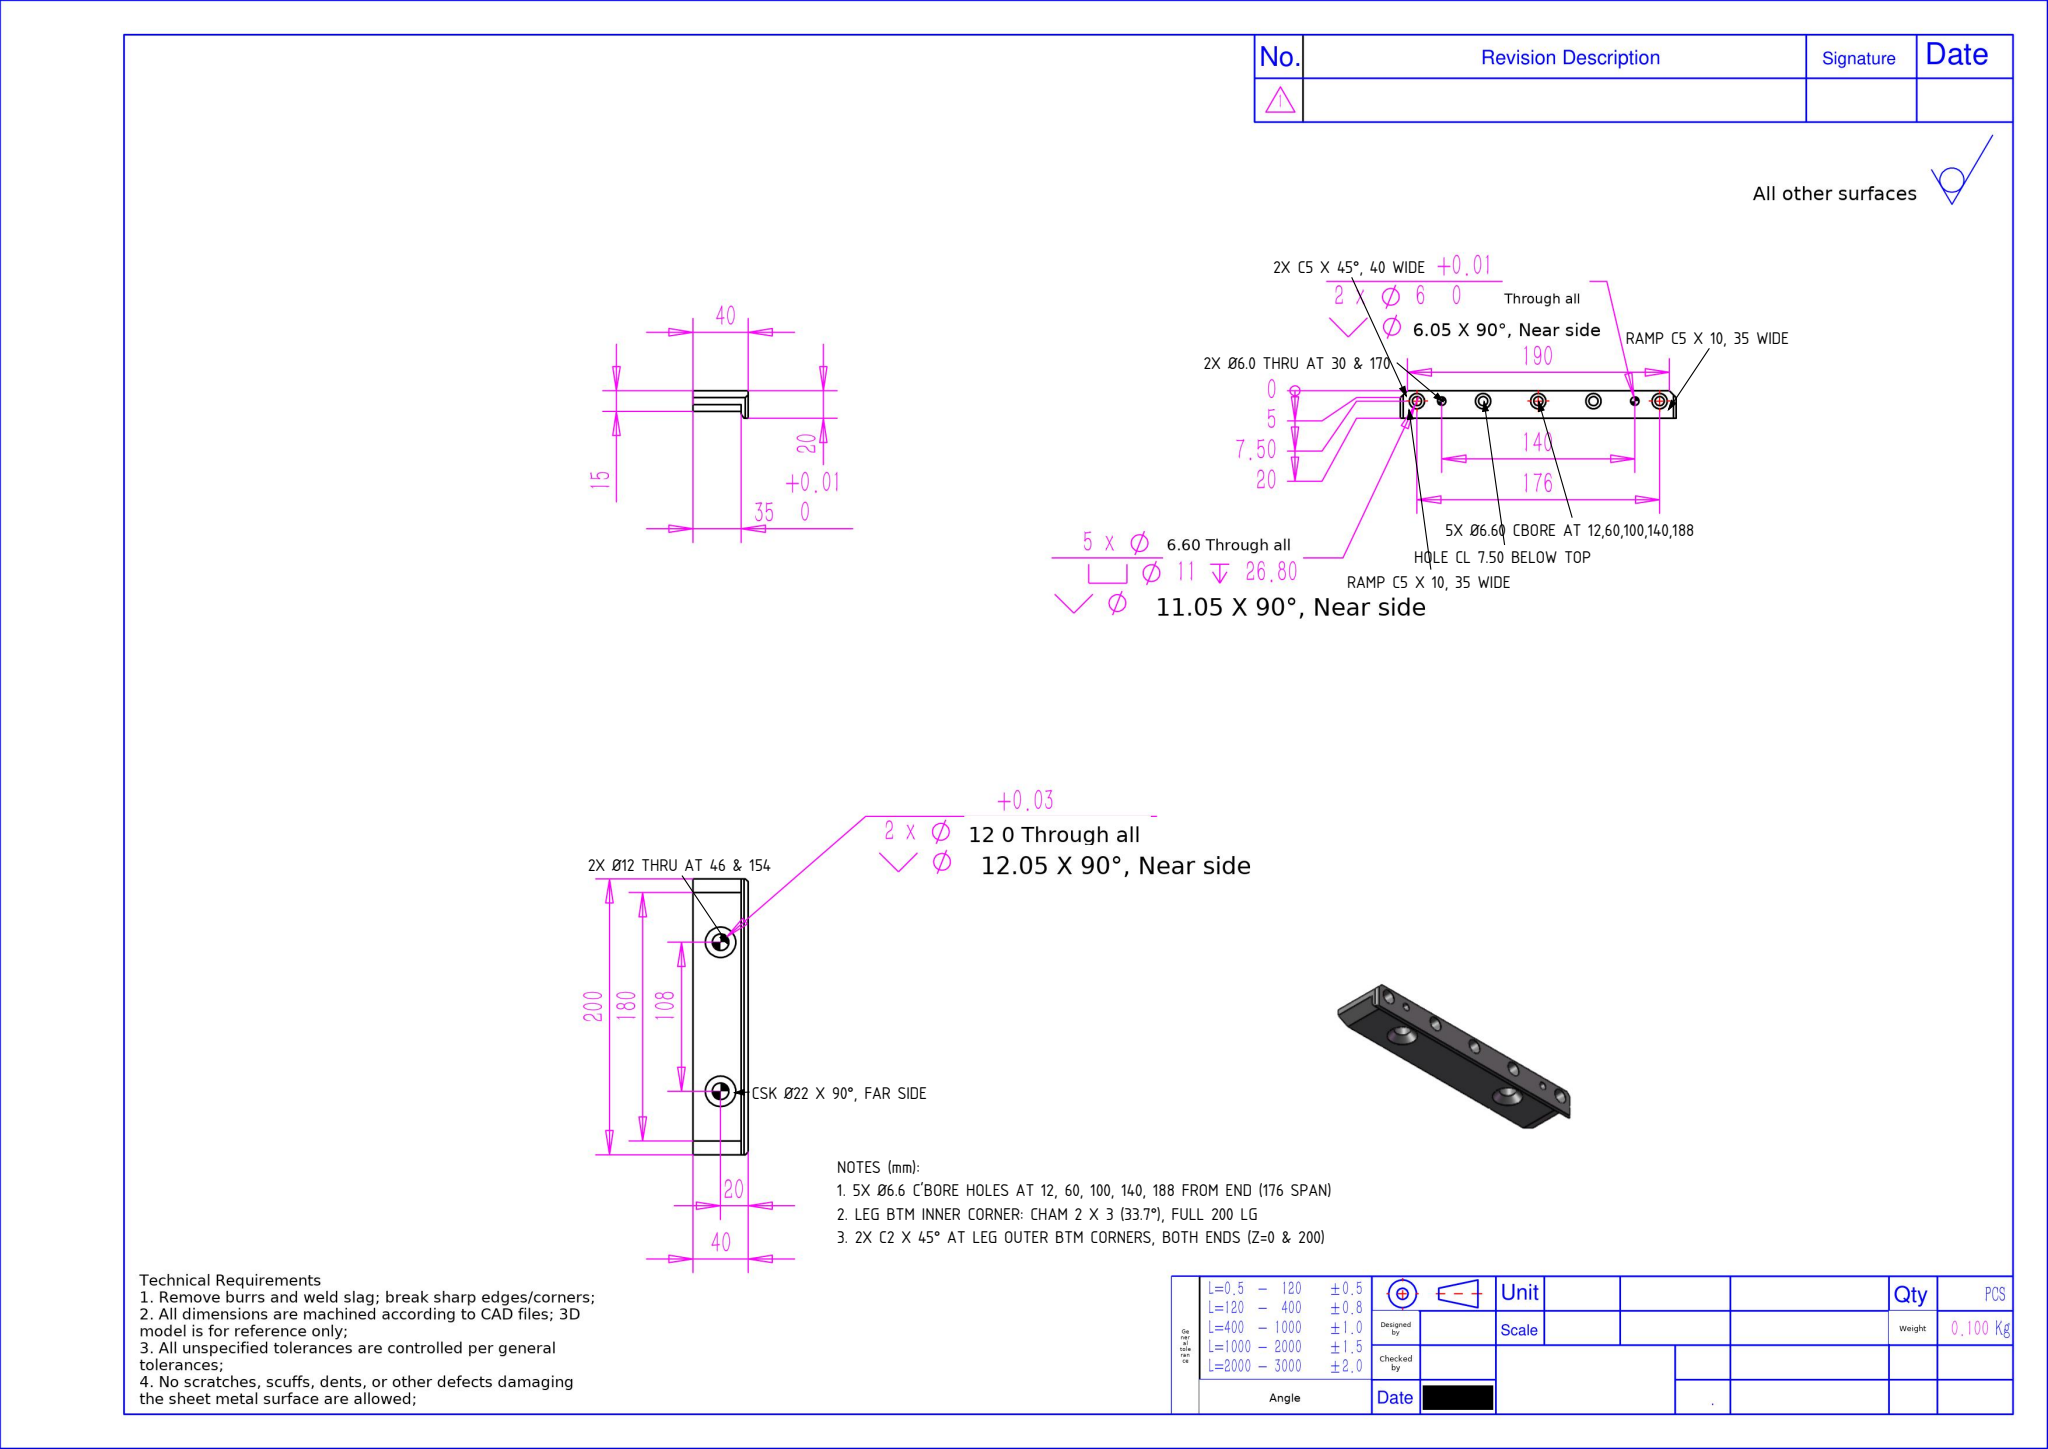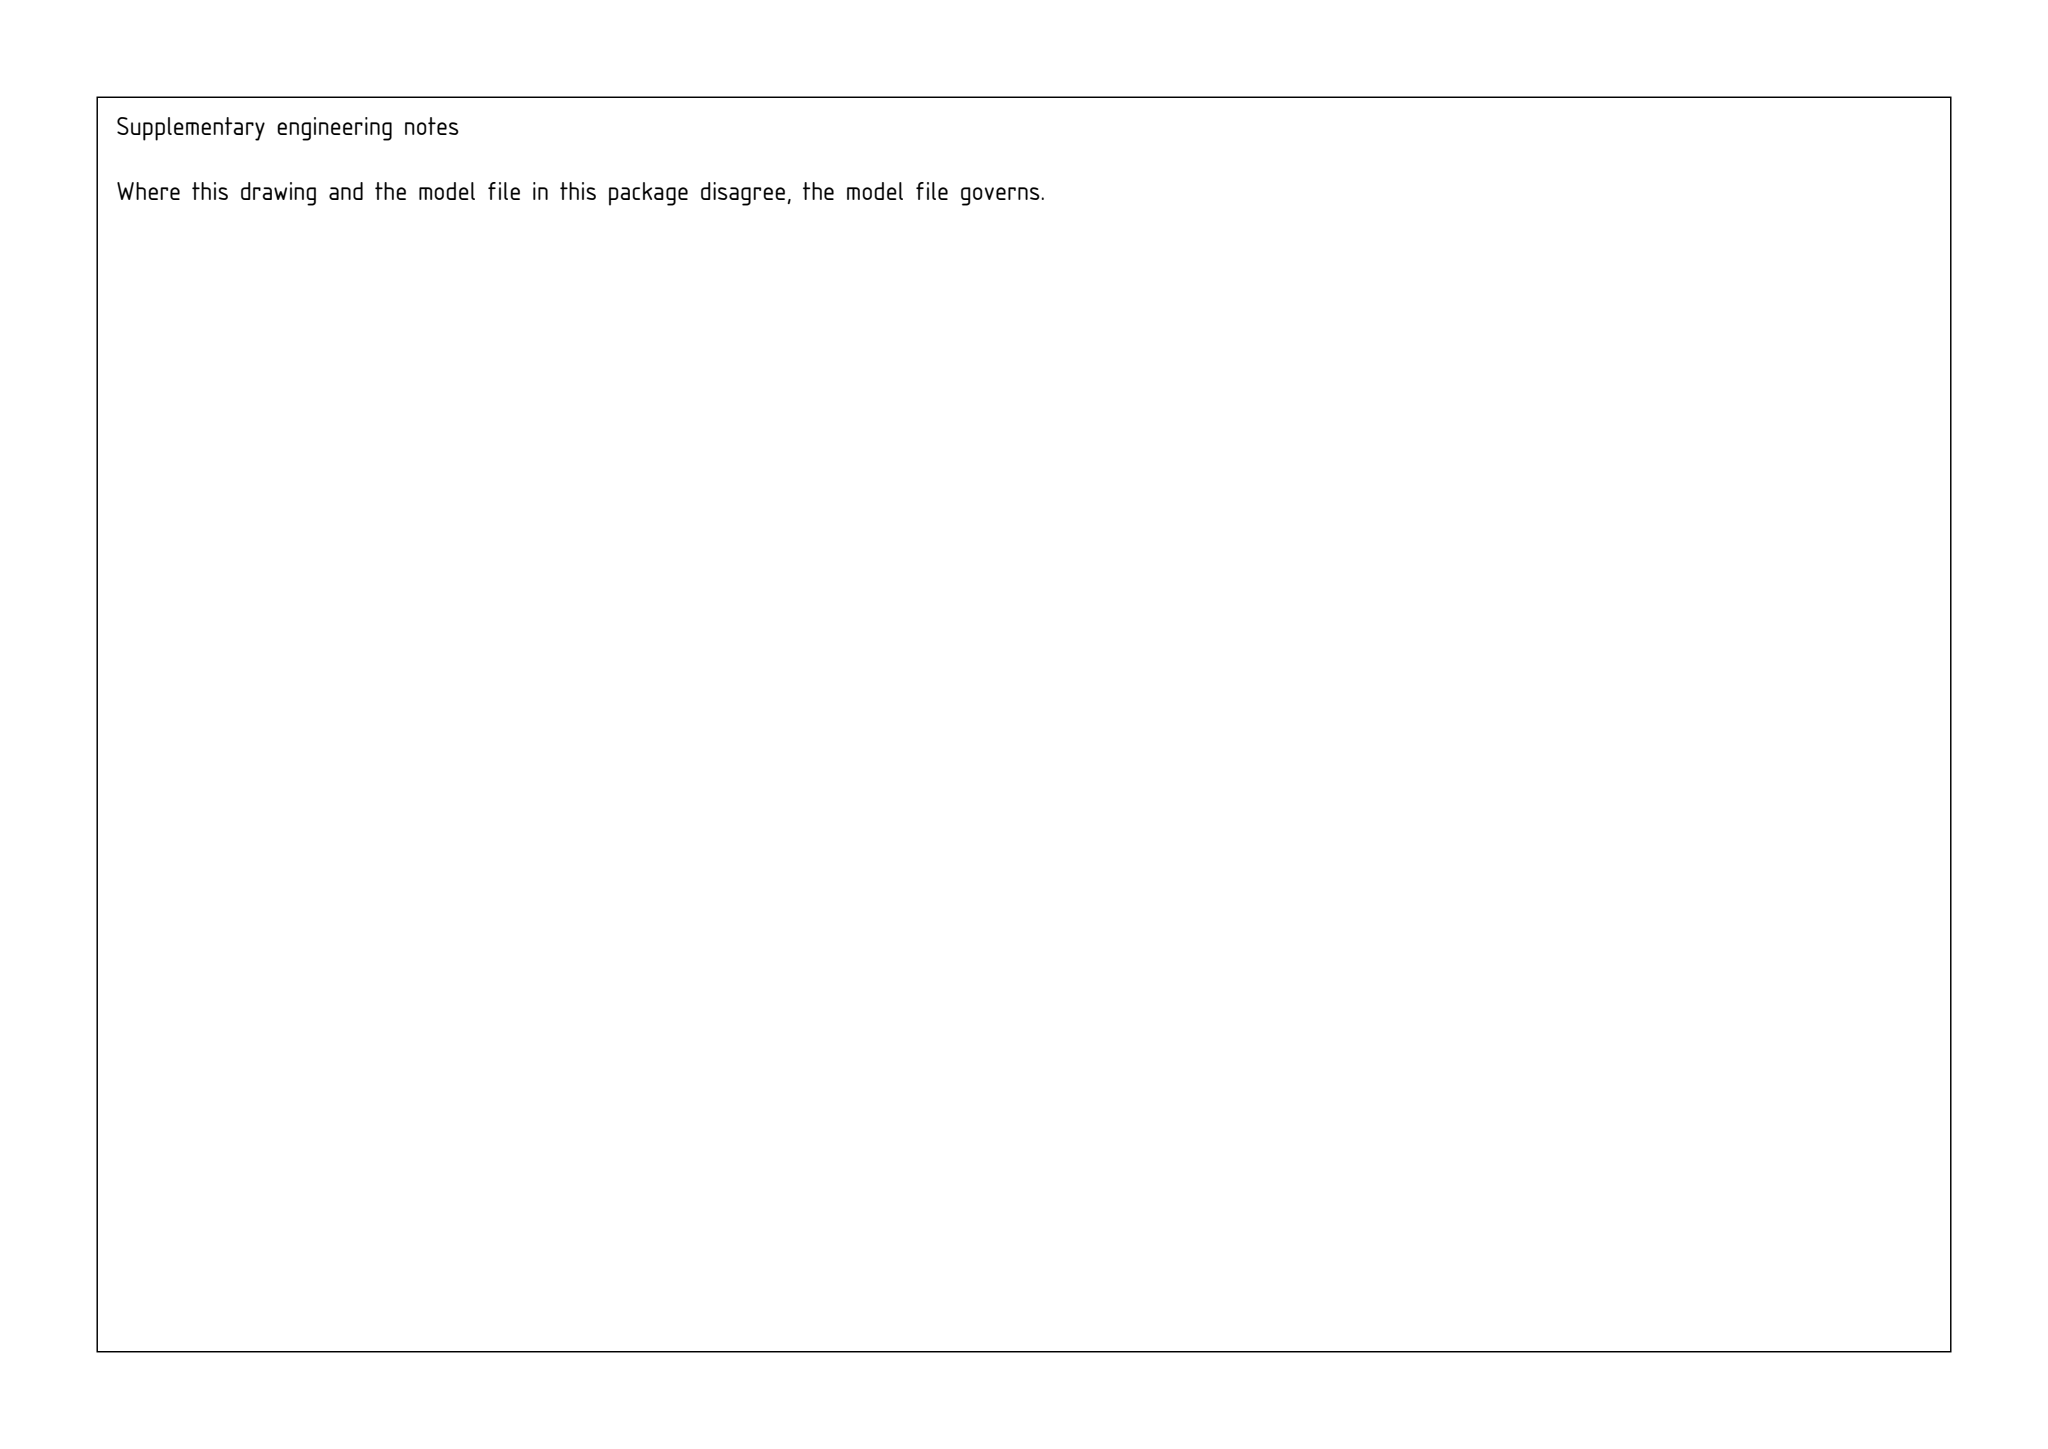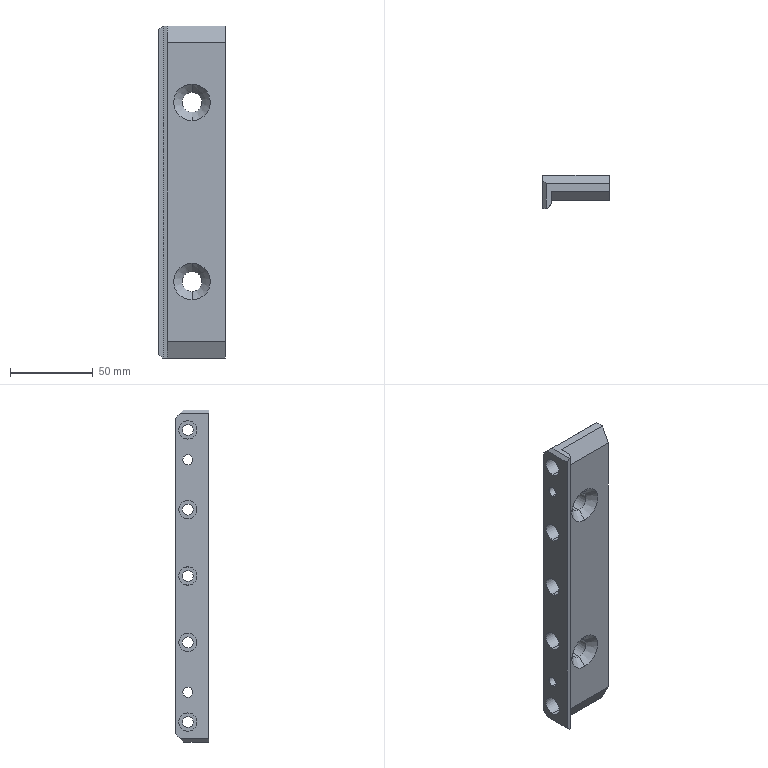Part | SolidWorks | mm | 1 solid | 70 faces | box 40 x 20 x 200 mm | volume 99736 mm3 | cylinder 28 | cone 22 | plane 20 | commonest cylinder face diameters 11 x10 6.6 x10 6 x4 12 x4
Drawing notes:
5X Ø6.60 CBORE HOLES AT 12, 60, 100, 140, 188 FROM LH END | from the solid: Ø6.6/Ø11 x-axis cyls at z = 12.0, 60.0, 100.0, 140.0, 188.0 of 200 lg
2X Ø6.0 THRU AT 30 & 170 FROM LH END | from the solid: Ø6.0 cyls, axis x, z = 30.0 and 170.0
ALL Ø6.60 & Ø6.0 HOLE CL 12.50 ABV BASE (7.50 BELOW TOP) | from the solid: all x-axis cyls at y = 12.5; y planes at 0, 5, 20
2X Ø12.0 THRU AT 46 & 154 FROM LH END, CL 20 FROM SIDE FACE | from the solid: Ø12.0 cyls, axis y, pos [20.0, null, 46.0] and [20.0, null, 154.0]
5X Ø6.6 C'BORE HOLES AT 12, 60, 100, 140, 188 FROM END (176 SPAN) | from the solid: Ø6.6/Ø11 bores at z=12,60,100,140,188; y=12.5; outer span 188-12=176
2X Ø12 THRU: ADD C'SINK Ø22 X 90°, FAR SIDE (FLANGE UNDERSIDE) | from the solid: cones 90°, ref_dia 12.0, from y=5 to y=10, size [11,5,22] at z=35 & 143
LEG BTM INNER CORNER: CHAM 2 X 3 (33.7°), FULL 200 LG | from the solid: inclined plane angles [33.7,56.3,90], from [3,0,0], size [2,3,200]
2X C2 X 45° AT LEG OUTER BTM CORNERS, BOTH ENDS (Z=0 & 200) | from the solid: inclined planes 45°, from [0,0,0] & [0,0,198], size [2,17,2]
2X C5 X 45° AT TOP EDGE OF BOTH END FACES, 40 WIDE | from the solid: inclined planes 45°, from [0,15,0] & [0,15,195], size [40,5,5]
FLANGE UNDERSIDE RAMP BOTH ENDS: 5 RISE X 10 RUN (26.6°), 35 WIDE | from the solid: inclined planes [90,26.6,63.4], from [5,5,0] & [5,5,190], size [35,5,10]
2X RAMP C5 X 10, 35 WIDE, BOTH ENDS OF 200 LG | from the solid: inclined_planes [90,26.6,63.4] at bbox_from [5,5,0] and [5,5,190], size [35,5,10] each
build123d program:
from build123d import *

# Parameters (mm, degrees)
BOSS_EXTRUDE1_DEPTH                            = 100
CHAMFER1_SIZE                                  = 2
M6_HEX_SOCKET_HEAD_CAP_SCREW_CBORE1_AT_2_COUNT = 2
M6_HEX_SOCKET_HEAD_CAP_SCREW_CBORE1_AT_2_PITCH = 88
M6_HEX_SOCKET_HEAD_CAP_SCREW_CBORE1_AT_3_COUNT = 2
M6_HEX_SOCKET_HEAD_CAP_SCREW_CBORE1_AT_3_PITCH = 176
M6_HEX_SOCKET_HEAD_CAP_SCREW_CBORE1_AT_4_COUNT = 2
M6_HEX_SOCKET_HEAD_CAP_SCREW_CBORE1_AT_4_PITCH = 48
M6_HEX_SOCKET_HEAD_CAP_SCREW_CBORE1_AT_5_COUNT = 2
M6_HEX_SOCKET_HEAD_CAP_SCREW_CBORE1_AT_5_PITCH = 128
F_12_0MM_DOWEL_PIN_HOLE1_D                     = 12
F_12_0MM_DOWEL_PIN_HOLE1_CSINK_D               = 12.05
F_12_0MM_DOWEL_PIN_HOLE1_CSINK_ANGLE           = 90
CHAMFER2_SIZE                                  = 5
CHAMFER2_SIZE2                                 = 10
F_6_0MM_DOWEL_PIN_HOLE1_D                      = 6
F_6_0MM_DOWEL_PIN_HOLE1_CSINK_D                = 6.05
F_6_0MM_DOWEL_PIN_HOLE1_CSINK_ANGLE            = 90
CHAMFER3_SIZE                                  = 10
CHAMFER3_SIZE2                                 = 5
CHAMFER4_SIZE                                  = 2
CHAMFER4_SIZE2                                 = 3
CHAMFER5_SIZE                                  = 5
CHAMFER6_SIZE                                  = 5


with BuildPart() as part:
    # Sketch1 → Boss-Extrude1 (new, symmetric)
    with BuildSketch(Plane.XY):
        Polygon((40, 0), (0, 0), (0, -20), (5, -20), (5, -15), (40, -15), align=None)
    extrude(amount=BOSS_EXTRUDE1_DEPTH, both=True)

    # Chamfer1
    chamfer1_edges = [part.edges().sort_by_distance(p)[0] for p in [
        (0, -10, -100),
        (0, -10, 100),
    ]]
    chamfer(chamfer1_edges, length=CHAMFER1_SIZE)

    # Sketch3 → M6 Hex Socket Head Cap Screw CBORE1 (revolve, cut)
    with BuildSketch(Plane(origin=(0, -7.5, -88), x_dir=(0, 0, 1), z_dir=(0, 1, 0))):
        Polygon((0, 0), (0, 40), (3.3, 40), (3.3, 26.8), (5.5, 26.8), (5.5, 0.025), (5.525, 0), align=None)
    m6_hex_socket_head_cap_screw_cbore1 = revolve(axis=Axis((-6.35, -7.5, -88), (1, 0, 0)), mode=Mode.SUBTRACT)

    # M6 Hex Socket Head Cap Screw CBORE1 at 2: M6 Hex Socket Head Cap Screw CBORE1 ×2
    with Locations(*[(0, 0, i * M6_HEX_SOCKET_HEAD_CAP_SCREW_CBORE1_AT_2_PITCH) for i in range(1, M6_HEX_SOCKET_HEAD_CAP_SCREW_CBORE1_AT_2_COUNT)]):
        add(m6_hex_socket_head_cap_screw_cbore1, mode=Mode.SUBTRACT)

    # M6 Hex Socket Head Cap Screw CBORE1 at 3: M6 Hex Socket Head Cap Screw CBORE1 ×2
    with Locations(*[(0, 0, i * M6_HEX_SOCKET_HEAD_CAP_SCREW_CBORE1_AT_3_PITCH) for i in range(1, M6_HEX_SOCKET_HEAD_CAP_SCREW_CBORE1_AT_3_COUNT)]):
        add(m6_hex_socket_head_cap_screw_cbore1, mode=Mode.SUBTRACT)

    # M6 Hex Socket Head Cap Screw CBORE1 at 4: M6 Hex Socket Head Cap Screw CBORE1 ×2
    with Locations(*[(0, 0, i * M6_HEX_SOCKET_HEAD_CAP_SCREW_CBORE1_AT_4_PITCH) for i in range(1, M6_HEX_SOCKET_HEAD_CAP_SCREW_CBORE1_AT_4_COUNT)]):
        add(m6_hex_socket_head_cap_screw_cbore1, mode=Mode.SUBTRACT)

    # M6 Hex Socket Head Cap Screw CBORE1 at 5: M6 Hex Socket Head Cap Screw CBORE1 ×2
    with Locations(*[(0, 0, i * M6_HEX_SOCKET_HEAD_CAP_SCREW_CBORE1_AT_5_PITCH) for i in range(1, M6_HEX_SOCKET_HEAD_CAP_SCREW_CBORE1_AT_5_COUNT)]):
        add(m6_hex_socket_head_cap_screw_cbore1, mode=Mode.SUBTRACT)

    # 12.0mm Dowel Pin Hole1 (through all)
    with Locations(Plane(origin=(0, 0, 0), x_dir=(1, 0, 0), z_dir=(0, 1, 0))):
        with Locations((20, 54)):
            f_12_0mm_dowel_pin_hole1 = CounterSinkHole(F_12_0MM_DOWEL_PIN_HOLE1_D / 2, F_12_0MM_DOWEL_PIN_HOLE1_CSINK_D / 2, counter_sink_angle=F_12_0MM_DOWEL_PIN_HOLE1_CSINK_ANGLE)

    # Chamfer2
    chamfer2_edges = [part.edges().sort_by_distance(p)[0] for p in [
        (22.5, -15, 100),
    ]]
    chamfer2_side = [part.faces().sort_by_distance(p)[0] for p in [
        (20.551, -7.756, 100),
    ]]
    chamfer(chamfer2_edges, length=CHAMFER2_SIZE, length2=CHAMFER2_SIZE2, reference=chamfer2_side[0])

    # Mirror1: 12.0mm Dowel Pin Hole1 across plane
    add(f_12_0mm_dowel_pin_hole1.mirror(Plane.XY), mode=Mode.SUBTRACT)

    # 6.0mm Dowel Pin Hole1 (through all)
    with Locations(Plane.ZY):
        with Locations((-70, -7.5), (70, -7.5)):
            CounterSinkHole(F_6_0MM_DOWEL_PIN_HOLE1_D / 2, F_6_0MM_DOWEL_PIN_HOLE1_CSINK_D / 2, counter_sink_angle=F_6_0MM_DOWEL_PIN_HOLE1_CSINK_ANGLE)

    # Chamfer3
    chamfer3_edges = [part.edges().sort_by_distance(p)[0] for p in [
        (22.5, -15, -100),
    ]]
    chamfer3_side = [part.faces().sort_by_distance(p)[0] for p in [
        (22.588, -15, -5.176),
    ]]
    chamfer(chamfer3_edges, length=CHAMFER3_SIZE, length2=CHAMFER3_SIZE2, reference=chamfer3_side[0])

    # Chamfer4
    chamfer4_edges = [part.edges().sort_by_distance(p)[0] for p in [
        (5, -20, 0),
    ]]
    chamfer4_side = [part.faces().sort_by_distance(p)[0] for p in [
        (2.507, -20, 0),
    ]]
    chamfer(chamfer4_edges, length=CHAMFER4_SIZE, length2=CHAMFER4_SIZE2, reference=chamfer4_side[0])

    # Chamfer5
    chamfer5_edges = [part.edges().sort_by_distance(p)[0] for p in [
        (26, -15, 54),
        (26, -15, -54),
    ]]
    chamfer(chamfer5_edges, length=CHAMFER5_SIZE)

    # Chamfer6
    chamfer6_edges = [part.edges().sort_by_distance(p)[0] for p in [
        (21, 0, 100),
        (21, 0, -100),
    ]]
    chamfer(chamfer6_edges, length=CHAMFER6_SIZE)


solid = part.part